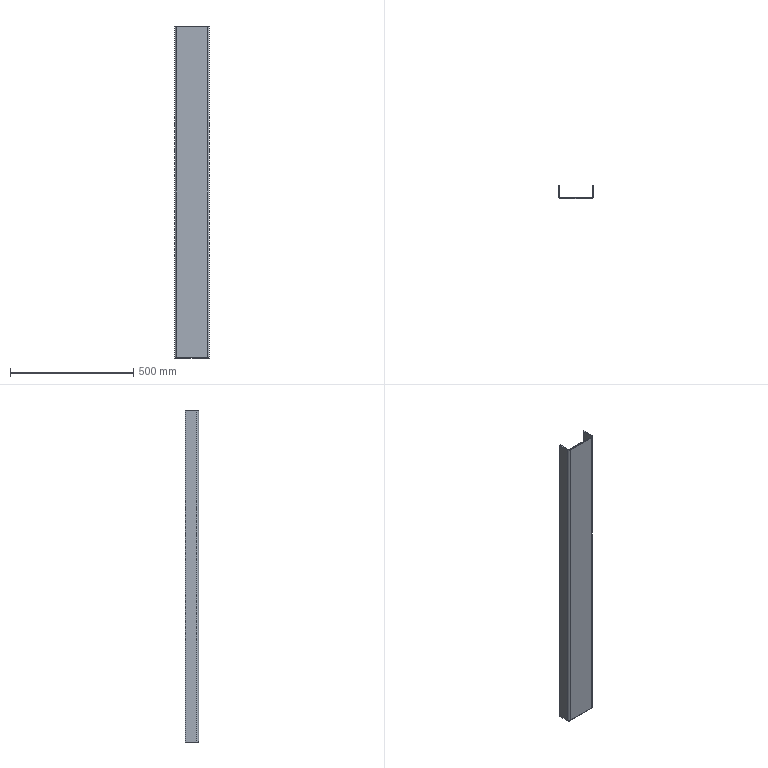Component | SolidWorks | LiftingVerticalBeamAssembly-2_LiftingVerticalBeam-1 | 1 solid | 26 faces | box 140 x 54 x 1345 mm | volume 1257606 mm3 | plane 22 | cylinder 4 | commonest cylinder face diameters 10 x2 18 x2 | material Plain Carbon Steel
STEP:
#1=CARTESIAN_POINT('',(14.893,-1.27,79.625));
#2=VERTEX_POINT('',#1);
#3=CARTESIAN_POINT('',(14.661,-1.27,79.625));
#4=VERTEX_POINT('',#3);
#5=CARTESIAN_POINT('',(14.539,-1.27,79.625));
#6=DIRECTION('',(-1.,0.,0.));
#7=VECTOR('',#6,39.37);
#8=LINE('',#5,#7);
#9=EDGE_CURVE('',#2,#4,#8,.T.);
#10=ORIENTED_EDGE('',*,*,#9,.F.);
#11=CARTESIAN_POINT('',(14.893,-1.199,79.625));
#12=VERTEX_POINT('',#11);
#13=CARTESIAN_POINT('',(14.893,-1.199,79.625));
#14=DIRECTION('',(0.,-1.,0.));
#15=VECTOR('',#14,39.37);
#16=LINE('',#13,#15);
#17=EDGE_CURVE('',#12,#2,#16,.T.);
#18=ORIENTED_EDGE('',*,*,#17,.F.);
#19=CARTESIAN_POINT('',(14.696,-1.002,79.625));
#20=VERTEX_POINT('',#19);
#21=CARTESIAN_POINT('',(14.893,-1.002,79.625));
#22=DIRECTION('',(0.,0.,1.));
#23=DIRECTION('',(1.,0.,0.));
#24=AXIS2_PLACEMENT_3D('',#21,#22,#23);
#25=CIRCLE('',#24,0.1969);
#26=EDGE_CURVE('',#20,#12,#25,.T.);
#27=ORIENTED_EDGE('',*,*,#26,.F.);
#28=CARTESIAN_POINT('',(14.539,-1.002,79.625));
#29=VERTEX_POINT('',#28);
#30=CARTESIAN_POINT('',(14.539,-1.002,79.625));
#31=DIRECTION('',(1.,0.,0.));
#32=VECTOR('',#31,39.37);
#33=LINE('',#30,#32);
#34=EDGE_CURVE('',#29,#20,#33,.T.);
#35=ORIENTED_EDGE('',*,*,#34,.F.);
#36=CARTESIAN_POINT('',(14.893,-1.002,79.625));
#37=DIRECTION('',(0.,0.,1.));
#38=DIRECTION('',(-1.,0.,0.));
#39=AXIS2_PLACEMENT_3D('',#36,#37,#38);
#40=CIRCLE('',#39,0.3543);
#41=EDGE_CURVE('',#29,#4,#40,.T.);
#42=ORIENTED_EDGE('',*,*,#41,.T.);
#43=EDGE_LOOP('',(#10,#18,#27,#35,#42));
#44=FACE_OUTER_BOUND('',#43,.T.);
#45=CARTESIAN_POINT('',(14.539,-1.002,79.625));
#46=DIRECTION('',(0.,0.,1.));
#47=DIRECTION('',(1.,0.,0.));
#48=AXIS2_PLACEMENT_3D('',#45,#46,#47);
#49=PLANE('',#48);
#50=ADVANCED_FACE('',(#44),#49,.T.);
#51=CARTESIAN_POINT('',(14.539,0.7696,79.625));
#52=VERTEX_POINT('',#51);
#53=CARTESIAN_POINT('',(14.539,0.7696,79.625));
#54=DIRECTION('',(0.,-1.,0.));
#55=VECTOR('',#54,39.37);
#56=LINE('',#53,#55);
#57=EDGE_CURVE('',#52,#29,#56,.T.);
#58=ORIENTED_EDGE('',*,*,#57,.T.);
#59=ORIENTED_EDGE('',*,*,#34,.T.);
#60=CARTESIAN_POINT('',(14.696,0.7696,79.625));
#61=VERTEX_POINT('',#60);
#62=CARTESIAN_POINT('',(14.696,0.7696,79.625));
#63=DIRECTION('',(0.,-1.,0.));
#64=VECTOR('',#63,39.37);
#65=LINE('',#62,#64);
#66=EDGE_CURVE('',#61,#20,#65,.T.);
#67=ORIENTED_EDGE('',*,*,#66,.F.);
#68=CARTESIAN_POINT('',(14.539,0.7696,79.625));
#69=DIRECTION('',(1.,0.,0.));
#70=VECTOR('',#69,39.37);
#71=LINE('',#68,#70);
#72=EDGE_CURVE('',#52,#61,#71,.T.);
#73=ORIENTED_EDGE('',*,*,#72,.F.);
#74=EDGE_LOOP('',(#58,#59,#67,#73));
#75=FACE_OUTER_BOUND('',#74,.T.);
#76=CARTESIAN_POINT('',(14.893,-1.199,79.625));
#77=DIRECTION('',(0.,0.,1.));
#78=DIRECTION('',(1.,0.,0.));
#79=AXIS2_PLACEMENT_3D('',#76,#77,#78);
#80=PLANE('',#79);
#81=ADVANCED_FACE('',(#75),#80,.T.);
#82=CARTESIAN_POINT('',(14.661,-1.27,26.672));
#83=VERTEX_POINT('',#82);
#84=CARTESIAN_POINT('',(14.893,-1.27,26.672));
#85=VERTEX_POINT('',#84);
#86=CARTESIAN_POINT('',(14.893,-1.27,26.672));
#87=DIRECTION('',(1.,0.,0.));
#88=VECTOR('',#87,39.37);
#89=LINE('',#86,#88);
#90=EDGE_CURVE('',#83,#85,#89,.T.);
#91=ORIENTED_EDGE('',*,*,#90,.F.);
#92=CARTESIAN_POINT('',(14.539,-1.002,26.672));
#93=VERTEX_POINT('',#92);
#94=CARTESIAN_POINT('',(14.893,-1.002,26.672));
#95=DIRECTION('',(0.,0.,1.));
#96=DIRECTION('',(-1.,0.,0.));
#97=AXIS2_PLACEMENT_3D('',#94,#95,#96);
#98=CIRCLE('',#97,0.3543);
#99=EDGE_CURVE('',#93,#83,#98,.T.);
#100=ORIENTED_EDGE('',*,*,#99,.F.);
#101=CARTESIAN_POINT('',(14.696,-1.002,26.672));
#102=VERTEX_POINT('',#101);
#103=CARTESIAN_POINT('',(14.696,-1.002,26.672));
#104=DIRECTION('',(-1.,0.,0.));
#105=VECTOR('',#104,39.37);
#106=LINE('',#103,#105);
#107=EDGE_CURVE('',#102,#93,#106,.T.);
#108=ORIENTED_EDGE('',*,*,#107,.F.);
#109=CARTESIAN_POINT('',(14.893,-1.199,26.672));
#110=VERTEX_POINT('',#109);
#111=CARTESIAN_POINT('',(14.893,-1.002,26.672));
#112=DIRECTION('',(0.,0.,1.));
#113=DIRECTION('',(1.,0.,0.));
#114=AXIS2_PLACEMENT_3D('',#111,#112,#113);
#115=CIRCLE('',#114,0.1969);
#116=EDGE_CURVE('',#102,#110,#115,.T.);
#117=ORIENTED_EDGE('',*,*,#116,.T.);
#118=CARTESIAN_POINT('',(14.893,-1.356,26.672));
#119=DIRECTION('',(0.,1.,0.));
#120=VECTOR('',#119,39.37);
#121=LINE('',#118,#120);
#122=EDGE_CURVE('',#85,#110,#121,.T.);
#123=ORIENTED_EDGE('',*,*,#122,.F.);
#124=EDGE_LOOP('',(#91,#100,#108,#117,#123));
#125=FACE_OUTER_BOUND('',#124,.T.);
#126=CARTESIAN_POINT('',(14.893,-1.356,26.672));
#127=DIRECTION('',(0.,0.,-1.));
#128=DIRECTION('',(-1.,0.,0.));
#129=AXIS2_PLACEMENT_3D('',#126,#127,#128);
#130=PLANE('',#129);
#131=ADVANCED_FACE('',(#125),#130,.T.);
#132=CARTESIAN_POINT('',(19.696,-1.27,26.672));
#133=VERTEX_POINT('',#132);
#134=CARTESIAN_POINT('',(14.696,-1.27,26.672));
#135=DIRECTION('',(1.,0.,0.));
#136=VECTOR('',#135,39.37);
#137=LINE('',#134,#136);
#138=EDGE_CURVE('',#85,#133,#137,.T.);
#139=ORIENTED_EDGE('',*,*,#138,.F.);
#140=ORIENTED_EDGE('',*,*,#122,.T.);
#141=CARTESIAN_POINT('',(19.696,-1.199,26.672));
#142=VERTEX_POINT('',#141);
#143=CARTESIAN_POINT('',(14.539,-1.199,26.672));
#144=DIRECTION('',(1.,0.,0.));
#145=VECTOR('',#144,39.37);
#146=LINE('',#143,#145);
#147=EDGE_CURVE('',#110,#142,#146,.T.);
#148=ORIENTED_EDGE('',*,*,#147,.T.);
#149=CARTESIAN_POINT('',(19.696,-1.199,26.672));
#150=DIRECTION('',(0.,-1.,0.));
#151=VECTOR('',#150,39.37);
#152=LINE('',#149,#151);
#153=EDGE_CURVE('',#142,#133,#152,.T.);
#154=ORIENTED_EDGE('',*,*,#153,.T.);
#155=EDGE_LOOP('',(#139,#140,#148,#154));
#156=FACE_OUTER_BOUND('',#155,.T.);
#157=CARTESIAN_POINT('',(14.696,-1.002,26.672));
#158=DIRECTION('',(0.,0.,-1.));
#159=DIRECTION('',(-1.,0.,0.));
#160=AXIS2_PLACEMENT_3D('',#157,#158,#159);
#161=PLANE('',#160);
#162=ADVANCED_FACE('',(#156),#161,.T.);
#163=CARTESIAN_POINT('',(19.929,-1.27,79.625));
#164=VERTEX_POINT('',#163);
#165=CARTESIAN_POINT('',(19.696,-1.27,79.625));
#166=VERTEX_POINT('',#165);
#167=CARTESIAN_POINT('',(19.696,-1.27,79.625));
#168=DIRECTION('',(-1.,0.,0.));
#169=VECTOR('',#168,39.37);
#170=LINE('',#167,#169);
#171=EDGE_CURVE('',#164,#166,#170,.T.);
#172=ORIENTED_EDGE('',*,*,#171,.F.);
#173=CARTESIAN_POINT('',(20.051,-1.002,79.625));
#174=VERTEX_POINT('',#173);
#175=CARTESIAN_POINT('',(19.696,-1.002,79.625));
#176=DIRECTION('',(0.,0.,1.));
#177=DIRECTION('',(-1.,-0.,0.));
#178=AXIS2_PLACEMENT_3D('',#175,#176,#177);
#179=CIRCLE('',#178,0.3543);
#180=EDGE_CURVE('',#164,#174,#179,.T.);
#181=ORIENTED_EDGE('',*,*,#180,.T.);
#182=CARTESIAN_POINT('',(19.893,-1.002,79.625));
#183=VERTEX_POINT('',#182);
#184=CARTESIAN_POINT('',(19.893,-1.002,79.625));
#185=DIRECTION('',(1.,0.,0.));
#186=VECTOR('',#185,39.37);
#187=LINE('',#184,#186);
#188=EDGE_CURVE('',#183,#174,#187,.T.);
#189=ORIENTED_EDGE('',*,*,#188,.F.);
#190=CARTESIAN_POINT('',(19.696,-1.199,79.625));
#191=VERTEX_POINT('',#190);
#192=CARTESIAN_POINT('',(19.696,-1.002,79.625));
#193=DIRECTION('',(0.,0.,1.));
#194=DIRECTION('',(1.,0.,0.));
#195=AXIS2_PLACEMENT_3D('',#192,#193,#194);
#196=CIRCLE('',#195,0.1969);
#197=EDGE_CURVE('',#191,#183,#196,.T.);
#198=ORIENTED_EDGE('',*,*,#197,.F.);
#199=CARTESIAN_POINT('',(19.696,-1.356,79.625));
#200=DIRECTION('',(0.,1.,0.));
#201=VECTOR('',#200,39.37);
#202=LINE('',#199,#201);
#203=EDGE_CURVE('',#166,#191,#202,.T.);
#204=ORIENTED_EDGE('',*,*,#203,.F.);
#205=EDGE_LOOP('',(#172,#181,#189,#198,#204));
#206=FACE_OUTER_BOUND('',#205,.T.);
#207=CARTESIAN_POINT('',(19.696,-1.356,79.625));
#208=DIRECTION('',(0.,0.,1.));
#209=DIRECTION('',(1.,0.,0.));
#210=AXIS2_PLACEMENT_3D('',#207,#208,#209);
#211=PLANE('',#210);
#212=ADVANCED_FACE('',(#206),#211,.T.);
#213=CARTESIAN_POINT('',(19.893,-1.27,79.625));
#214=DIRECTION('',(-1.,0.,0.));
#215=VECTOR('',#214,39.37);
#216=LINE('',#213,#215);
#217=EDGE_CURVE('',#166,#2,#216,.T.);
#218=ORIENTED_EDGE('',*,*,#217,.F.);
#219=ORIENTED_EDGE('',*,*,#203,.T.);
#220=CARTESIAN_POINT('',(14.539,-1.199,79.625));
#221=DIRECTION('',(1.,0.,0.));
#222=VECTOR('',#221,39.37);
#223=LINE('',#220,#222);
#224=EDGE_CURVE('',#12,#191,#223,.T.);
#225=ORIENTED_EDGE('',*,*,#224,.F.);
#226=ORIENTED_EDGE('',*,*,#17,.T.);
#227=EDGE_LOOP('',(#218,#219,#225,#226));
#228=FACE_OUTER_BOUND('',#227,.T.);
#229=CARTESIAN_POINT('',(19.893,-1.002,79.625));
#230=DIRECTION('',(0.,0.,1.));
#231=DIRECTION('',(1.,0.,0.));
#232=AXIS2_PLACEMENT_3D('',#229,#230,#231);
#233=PLANE('',#232);
#234=ADVANCED_FACE('',(#228),#233,.T.);
#235=CARTESIAN_POINT('',(19.929,-1.27,26.672));
#236=VERTEX_POINT('',#235);
#237=CARTESIAN_POINT('',(20.051,-1.27,26.672));
#238=DIRECTION('',(1.,0.,0.));
#239=VECTOR('',#238,39.37);
#240=LINE('',#237,#239);
#241=EDGE_CURVE('',#133,#236,#240,.T.);
#242=ORIENTED_EDGE('',*,*,#241,.F.);
#243=ORIENTED_EDGE('',*,*,#153,.F.);
#244=CARTESIAN_POINT('',(19.893,-1.002,26.672));
#245=VERTEX_POINT('',#244);
#246=CARTESIAN_POINT('',(19.696,-1.002,26.672));
#247=DIRECTION('',(0.,0.,1.));
#248=DIRECTION('',(1.,0.,0.));
#249=AXIS2_PLACEMENT_3D('',#246,#247,#248);
#250=CIRCLE('',#249,0.1969);
#251=EDGE_CURVE('',#142,#245,#250,.T.);
#252=ORIENTED_EDGE('',*,*,#251,.T.);
#253=CARTESIAN_POINT('',(20.051,-1.002,26.672));
#254=VERTEX_POINT('',#253);
#255=CARTESIAN_POINT('',(20.051,-1.002,26.672));
#256=DIRECTION('',(-1.,0.,0.));
#257=VECTOR('',#256,39.37);
#258=LINE('',#255,#257);
#259=EDGE_CURVE('',#254,#245,#258,.T.);
#260=ORIENTED_EDGE('',*,*,#259,.F.);
#261=CARTESIAN_POINT('',(19.696,-1.002,26.672));
#262=DIRECTION('',(0.,0.,1.));
#263=DIRECTION('',(-1.,-0.,0.));
#264=AXIS2_PLACEMENT_3D('',#261,#262,#263);
#265=CIRCLE('',#264,0.3543);
#266=EDGE_CURVE('',#236,#254,#265,.T.);
#267=ORIENTED_EDGE('',*,*,#266,.F.);
#268=EDGE_LOOP('',(#242,#243,#252,#260,#267));
#269=FACE_OUTER_BOUND('',#268,.T.);
#270=CARTESIAN_POINT('',(20.051,-1.002,26.672));
#271=DIRECTION('',(0.,0.,-1.));
#272=DIRECTION('',(-1.,0.,0.));
#273=AXIS2_PLACEMENT_3D('',#270,#271,#272);
#274=PLANE('',#273);
#275=ADVANCED_FACE('',(#269),#274,.T.);
#276=CARTESIAN_POINT('',(20.051,0.7696,26.672));
#277=VERTEX_POINT('',#276);
#278=CARTESIAN_POINT('',(20.051,-1.356,26.672));
#279=DIRECTION('',(0.,1.,0.));
#280=VECTOR('',#279,39.37);
#281=LINE('',#278,#280);
#282=EDGE_CURVE('',#254,#277,#281,.T.);
#283=ORIENTED_EDGE('',*,*,#282,.F.);
#284=ORIENTED_EDGE('',*,*,#259,.T.);
#285=CARTESIAN_POINT('',(19.893,0.7696,26.672));
#286=VERTEX_POINT('',#285);
#287=CARTESIAN_POINT('',(19.893,-1.356,26.672));
#288=DIRECTION('',(0.,1.,0.));
#289=VECTOR('',#288,39.37);
#290=LINE('',#287,#289);
#291=EDGE_CURVE('',#245,#286,#290,.T.);
#292=ORIENTED_EDGE('',*,*,#291,.T.);
#293=CARTESIAN_POINT('',(19.893,0.7696,26.672));
#294=DIRECTION('',(1.,0.,0.));
#295=VECTOR('',#294,39.37);
#296=LINE('',#293,#295);
#297=EDGE_CURVE('',#286,#277,#296,.T.);
#298=ORIENTED_EDGE('',*,*,#297,.T.);
#299=EDGE_LOOP('',(#283,#284,#292,#298));
#300=FACE_OUTER_BOUND('',#299,.T.);
#301=CARTESIAN_POINT('',(19.696,-1.199,26.672));
#302=DIRECTION('',(0.,0.,-1.));
#303=DIRECTION('',(-1.,0.,0.));
#304=AXIS2_PLACEMENT_3D('',#301,#302,#303);
#305=PLANE('',#304);
#306=ADVANCED_FACE('',(#300),#305,.T.);
#307=ORIENTED_EDGE('',*,*,#282,.T.);
#308=CARTESIAN_POINT('',(20.051,0.7696,79.625));
#309=VERTEX_POINT('',#308);
#310=CARTESIAN_POINT('',(20.051,0.7696,79.625));
#311=DIRECTION('',(0.,0.,-1.));
#312=VECTOR('',#311,39.37);
#313=LINE('',#310,#312);
#314=EDGE_CURVE('',#309,#277,#313,.T.);
#315=ORIENTED_EDGE('',*,*,#314,.F.);
#316=CARTESIAN_POINT('',(20.051,-1.356,79.625));
#317=DIRECTION('',(0.,1.,0.));
#318=VECTOR('',#317,39.37);
#319=LINE('',#316,#318);
#320=EDGE_CURVE('',#174,#309,#319,.T.);
#321=ORIENTED_EDGE('',*,*,#320,.F.);
#322=CARTESIAN_POINT('',(20.051,-1.002,79.625));
#323=DIRECTION('',(0.,0.,-1.));
#324=VECTOR('',#323,39.37);
#325=LINE('',#322,#324);
#326=EDGE_CURVE('',#174,#254,#325,.T.);
#327=ORIENTED_EDGE('',*,*,#326,.T.);
#328=EDGE_LOOP('',(#307,#315,#321,#327));
#329=FACE_OUTER_BOUND('',#328,.T.);
#330=CARTESIAN_POINT('',(20.051,-1.356,79.625));
#331=DIRECTION('',(-1.,0.,0.));
#332=DIRECTION('',(0.,0.,1.));
#333=AXIS2_PLACEMENT_3D('',#330,#331,#332);
#334=PLANE('',#333);
#335=ADVANCED_FACE('',(#329),#334,.F.);
#336=ORIENTED_EDGE('',*,*,#297,.F.);
#337=CARTESIAN_POINT('',(19.893,0.7696,79.625));
#338=VERTEX_POINT('',#337);
#339=CARTESIAN_POINT('',(19.893,0.7696,79.625));
#340=DIRECTION('',(0.,0.,-1.));
#341=VECTOR('',#340,39.37);
#342=LINE('',#339,#341);
#343=EDGE_CURVE('',#338,#286,#342,.T.);
#344=ORIENTED_EDGE('',*,*,#343,.F.);
#345=CARTESIAN_POINT('',(19.893,0.7696,79.625));
#346=DIRECTION('',(1.,0.,0.));
#347=VECTOR('',#346,39.37);
#348=LINE('',#345,#347);
#349=EDGE_CURVE('',#338,#309,#348,.T.);
#350=ORIENTED_EDGE('',*,*,#349,.T.);
#351=ORIENTED_EDGE('',*,*,#314,.T.);
#352=EDGE_LOOP('',(#336,#344,#350,#351));
#353=FACE_OUTER_BOUND('',#352,.T.);
#354=CARTESIAN_POINT('',(19.893,0.7696,79.625));
#355=DIRECTION('',(0.,1.,0.));
#356=DIRECTION('',(0.,0.,1.));
#357=AXIS2_PLACEMENT_3D('',#354,#355,#356);
#358=PLANE('',#357);
#359=ADVANCED_FACE('',(#353),#358,.T.);
#360=ORIENTED_EDGE('',*,*,#291,.F.);
#361=CARTESIAN_POINT('',(19.893,-1.002,79.625));
#362=DIRECTION('',(0.,0.,-1.));
#363=VECTOR('',#362,39.37);
#364=LINE('',#361,#363);
#365=EDGE_CURVE('',#183,#245,#364,.T.);
#366=ORIENTED_EDGE('',*,*,#365,.F.);
#367=CARTESIAN_POINT('',(19.893,-1.356,79.625));
#368=DIRECTION('',(0.,1.,0.));
#369=VECTOR('',#368,39.37);
#370=LINE('',#367,#369);
#371=EDGE_CURVE('',#183,#338,#370,.T.);
#372=ORIENTED_EDGE('',*,*,#371,.T.);
#373=ORIENTED_EDGE('',*,*,#343,.T.);
#374=EDGE_LOOP('',(#360,#366,#372,#373));
#375=FACE_OUTER_BOUND('',#374,.T.);
#376=CARTESIAN_POINT('',(19.893,-1.356,79.625));
#377=DIRECTION('',(-1.,0.,0.));
#378=DIRECTION('',(0.,0.,1.));
#379=AXIS2_PLACEMENT_3D('',#376,#377,#378);
#380=PLANE('',#379);
#381=ADVANCED_FACE('',(#375),#380,.T.);
#382=ORIENTED_EDGE('',*,*,#251,.F.);
#383=CARTESIAN_POINT('',(19.696,-1.199,79.625));
#384=DIRECTION('',(0.,0.,-1.));
#385=VECTOR('',#384,39.37);
#386=LINE('',#383,#385);
#387=EDGE_CURVE('',#191,#142,#386,.T.);
#388=ORIENTED_EDGE('',*,*,#387,.F.);
#389=ORIENTED_EDGE('',*,*,#197,.T.);
#390=ORIENTED_EDGE('',*,*,#365,.T.);
#391=EDGE_LOOP('',(#382,#388,#389,#390));
#392=FACE_OUTER_BOUND('',#391,.T.);
#393=CARTESIAN_POINT('',(19.696,-1.002,79.625));
#394=DIRECTION('',(0.,0.,-1.));
#395=DIRECTION('',(-1.,0.,0.));
#396=AXIS2_PLACEMENT_3D('',#393,#394,#395);
#397=CYLINDRICAL_SURFACE('',#396,0.1969);
#398=ADVANCED_FACE('',(#392),#397,.F.);
#399=ORIENTED_EDGE('',*,*,#147,.F.);
#400=CARTESIAN_POINT('',(14.893,-1.199,79.625));
#401=DIRECTION('',(0.,0.,-1.));
#402=VECTOR('',#401,39.37);
#403=LINE('',#400,#402);
#404=EDGE_CURVE('',#12,#110,#403,.T.);
#405=ORIENTED_EDGE('',*,*,#404,.F.);
#406=ORIENTED_EDGE('',*,*,#224,.T.);
#407=ORIENTED_EDGE('',*,*,#387,.T.);
#408=EDGE_LOOP('',(#399,#405,#406,#407));
#409=FACE_OUTER_BOUND('',#408,.T.);
#410=CARTESIAN_POINT('',(14.539,-1.199,79.625));
#411=DIRECTION('',(0.,1.,0.));
#412=DIRECTION('',(0.,0.,1.));
#413=AXIS2_PLACEMENT_3D('',#410,#411,#412);
#414=PLANE('',#413);
#415=ADVANCED_FACE('',(#409),#414,.T.);
#416=ORIENTED_EDGE('',*,*,#116,.F.);
#417=CARTESIAN_POINT('',(14.696,-1.002,79.625));
#418=DIRECTION('',(0.,0.,-1.));
#419=VECTOR('',#418,39.37);
#420=LINE('',#417,#419);
#421=EDGE_CURVE('',#20,#102,#420,.T.);
#422=ORIENTED_EDGE('',*,*,#421,.F.);
#423=ORIENTED_EDGE('',*,*,#26,.T.);
#424=ORIENTED_EDGE('',*,*,#404,.T.);
#425=EDGE_LOOP('',(#416,#422,#423,#424));
#426=FACE_OUTER_BOUND('',#425,.T.);
#427=CARTESIAN_POINT('',(14.893,-1.002,79.625));
#428=DIRECTION('',(0.,0.,-1.));
#429=DIRECTION('',(-1.,0.,0.));
#430=AXIS2_PLACEMENT_3D('',#427,#428,#429);
#431=CYLINDRICAL_SURFACE('',#430,0.1969);
#432=ADVANCED_FACE('',(#426),#431,.F.);
#433=CARTESIAN_POINT('',(14.696,0.7696,26.672));
#434=VERTEX_POINT('',#433);
#435=CARTESIAN_POINT('',(14.696,0.7696,26.672));
#436=DIRECTION('',(0.,-1.,0.));
#437=VECTOR('',#436,39.37);
#438=LINE('',#435,#437);
#439=EDGE_CURVE('',#434,#102,#438,.T.);
#440=ORIENTED_EDGE('',*,*,#439,.F.);
#441=CARTESIAN_POINT('',(14.696,0.7696,79.625));
#442=DIRECTION('',(0.,0.,-1.));
#443=VECTOR('',#442,39.37);
#444=LINE('',#441,#443);
#445=EDGE_CURVE('',#61,#434,#444,.T.);
#446=ORIENTED_EDGE('',*,*,#445,.F.);
#447=ORIENTED_EDGE('',*,*,#66,.T.);
#448=ORIENTED_EDGE('',*,*,#421,.T.);
#449=EDGE_LOOP('',(#440,#446,#447,#448));
#450=FACE_OUTER_BOUND('',#449,.T.);
#451=CARTESIAN_POINT('',(14.696,0.7696,79.625));
#452=DIRECTION('',(1.,0.,0.));
#453=DIRECTION('',(-0.,1.,0.));
#454=AXIS2_PLACEMENT_3D('',#451,#452,#453);
#455=PLANE('',#454);
#456=ADVANCED_FACE('',(#450),#455,.T.);
#457=CARTESIAN_POINT('',(14.539,0.7696,26.672));
#458=VERTEX_POINT('',#457);
#459=CARTESIAN_POINT('',(14.539,0.7696,26.672));
#460=DIRECTION('',(1.,0.,0.));
#461=VECTOR('',#460,39.37);
#462=LINE('',#459,#461);
#463=EDGE_CURVE('',#458,#434,#462,.T.);
#464=ORIENTED_EDGE('',*,*,#463,.F.);
#465=CARTESIAN_POINT('',(14.539,0.7696,79.625));
#466=DIRECTION('',(0.,0.,-1.));
#467=VECTOR('',#466,39.37);
#468=LINE('',#465,#467);
#469=EDGE_CURVE('',#52,#458,#468,.T.);
#470=ORIENTED_EDGE('',*,*,#469,.F.);
#471=ORIENTED_EDGE('',*,*,#72,.T.);
#472=ORIENTED_EDGE('',*,*,#445,.T.);
#473=EDGE_LOOP('',(#464,#470,#471,#472));
#474=FACE_OUTER_BOUND('',#473,.T.);
#475=CARTESIAN_POINT('',(14.539,0.7696,79.625));
#476=DIRECTION('',(-0.,1.,0.));
#477=DIRECTION('',(-1.,-0.,0.));
#478=AXIS2_PLACEMENT_3D('',#475,#476,#477);
#479=PLANE('',#478);
#480=ADVANCED_FACE('',(#474),#479,.T.);
#481=CARTESIAN_POINT('',(14.539,0.7696,26.672));
#482=DIRECTION('',(0.,-1.,0.));
#483=VECTOR('',#482,39.37);
#484=LINE('',#481,#483);
#485=EDGE_CURVE('',#458,#93,#484,.T.);
#486=ORIENTED_EDGE('',*,*,#485,.T.);
#487=CARTESIAN_POINT('',(14.539,-1.002,79.625));
#488=DIRECTION('',(0.,0.,-1.));
#489=VECTOR('',#488,39.37);
#490=LINE('',#487,#489);
#491=EDGE_CURVE('',#29,#93,#490,.T.);
#492=ORIENTED_EDGE('',*,*,#491,.F.);
#493=ORIENTED_EDGE('',*,*,#57,.F.);
#494=ORIENTED_EDGE('',*,*,#469,.T.);
#495=EDGE_LOOP('',(#486,#492,#493,#494));
#496=FACE_OUTER_BOUND('',#495,.T.);
#497=CARTESIAN_POINT('',(14.539,0.7696,79.625));
#498=DIRECTION('',(1.,0.,0.));
#499=DIRECTION('',(-0.,1.,0.));
#500=AXIS2_PLACEMENT_3D('',#497,#498,#499);
#501=PLANE('',#500);
#502=ADVANCED_FACE('',(#496),#501,.F.);
#503=CARTESIAN_POINT('',(14.893,-1.356,79.538));
#504=VERTEX_POINT('',#503);
#505=CARTESIAN_POINT('',(14.893,-1.356,26.759));
#506=VERTEX_POINT('',#505);
#507=CARTESIAN_POINT('',(14.893,-1.356,79.625));
#508=DIRECTION('',(0.,0.,-1.));
#509=VECTOR('',#508,39.37);
#510=LINE('',#507,#509);
#511=EDGE_CURVE('',#504,#506,#510,.T.);
#512=ORIENTED_EDGE('',*,*,#511,.F.);
#513=CARTESIAN_POINT('',(14.661,-1.27,79.538));
#514=VERTEX_POINT('',#513);
#515=CARTESIAN_POINT('',(14.893,-1.002,79.538));
#516=DIRECTION('',(0.,0.,-1.));
#517=DIRECTION('',(-1.,0.,0.));
#518=AXIS2_PLACEMENT_3D('',#515,#516,#517);
#519=CIRCLE('',#518,0.3543);
#520=EDGE_CURVE('',#504,#514,#519,.T.);
#521=ORIENTED_EDGE('',*,*,#520,.T.);
#522=CARTESIAN_POINT('',(14.661,-1.27,79.625));
#523=DIRECTION('',(0.,0.,1.));
#524=VECTOR('',#523,39.37);
#525=LINE('',#522,#524);
#526=EDGE_CURVE('',#514,#4,#525,.T.);
#527=ORIENTED_EDGE('',*,*,#526,.T.);
#528=ORIENTED_EDGE('',*,*,#41,.F.);
#529=ORIENTED_EDGE('',*,*,#491,.T.);
#530=ORIENTED_EDGE('',*,*,#99,.T.);
#531=CARTESIAN_POINT('',(14.661,-1.27,26.759));
#532=VERTEX_POINT('',#531);
#533=CARTESIAN_POINT('',(14.661,-1.27,79.625));
#534=DIRECTION('',(0.,0.,1.));
#535=VECTOR('',#534,39.37);
#536=LINE('',#533,#535);
#537=EDGE_CURVE('',#83,#532,#536,.T.);
#538=ORIENTED_EDGE('',*,*,#537,.T.);
#539=CARTESIAN_POINT('',(14.893,-1.002,26.759));
#540=DIRECTION('',(0.,0.,1.));
#541=DIRECTION('',(1.,0.,0.));
#542=AXIS2_PLACEMENT_3D('',#539,#540,#541);
#543=CIRCLE('',#542,0.3543);
#544=EDGE_CURVE('',#532,#506,#543,.T.);
#545=ORIENTED_EDGE('',*,*,#544,.T.);
#546=EDGE_LOOP('',(#512,#521,#527,#528,#529,#530,#538,#545));
#547=FACE_OUTER_BOUND('',#546,.T.);
#548=CARTESIAN_POINT('',(14.893,-1.002,79.625));
#549=DIRECTION('',(0.,0.,-1.));
#550=DIRECTION('',(-1.,0.,0.));
#551=AXIS2_PLACEMENT_3D('',#548,#549,#550);
#552=CYLINDRICAL_SURFACE('',#551,0.3543);
#553=ADVANCED_FACE('',(#547),#552,.T.);
#554=CARTESIAN_POINT('',(19.696,-1.356,79.538));
#555=VERTEX_POINT('',#554);
#556=CARTESIAN_POINT('',(19.696,-1.356,26.759));
#557=VERTEX_POINT('',#556);
#558=CARTESIAN_POINT('',(19.696,-1.356,79.625));
#559=DIRECTION('',(0.,0.,-1.));
#560=VECTOR('',#559,39.37);
#561=LINE('',#558,#560);
#562=EDGE_CURVE('',#555,#557,#561,.T.);
#563=ORIENTED_EDGE('',*,*,#562,.F.);
#564=CARTESIAN_POINT('',(14.539,-1.356,79.538));
#565=DIRECTION('',(-1.,0.,0.));
#566=VECTOR('',#565,39.37);
#567=LINE('',#564,#566);
#568=EDGE_CURVE('',#555,#504,#567,.T.);
#569=ORIENTED_EDGE('',*,*,#568,.T.);
#570=ORIENTED_EDGE('',*,*,#511,.T.);
#571=CARTESIAN_POINT('',(14.539,-1.356,26.759));
#572=DIRECTION('',(1.,0.,0.));
#573=VECTOR('',#572,39.37);
#574=LINE('',#571,#573);
#575=EDGE_CURVE('',#506,#557,#574,.T.);
#576=ORIENTED_EDGE('',*,*,#575,.T.);
#577=EDGE_LOOP('',(#563,#569,#570,#576));
#578=FACE_OUTER_BOUND('',#577,.T.);
#579=CARTESIAN_POINT('',(14.539,-1.356,79.625));
#580=DIRECTION('',(0.,1.,0.));
#581=DIRECTION('',(0.,0.,1.));
#582=AXIS2_PLACEMENT_3D('',#579,#580,#581);
#583=PLANE('',#582);
#584=ADVANCED_FACE('',(#578),#583,.F.);
#585=CARTESIAN_POINT('',(19.929,-1.27,79.538));
#586=VERTEX_POINT('',#585);
#587=CARTESIAN_POINT('',(19.929,-1.27,79.625));
#588=DIRECTION('',(0.,0.,-1.));
#589=VECTOR('',#588,39.37);
#590=LINE('',#587,#589);
#591=EDGE_CURVE('',#164,#586,#590,.T.);
#592=ORIENTED_EDGE('',*,*,#591,.T.);
#593=CARTESIAN_POINT('',(19.696,-1.002,79.538));
#594=DIRECTION('',(0.,0.,-1.));
#595=DIRECTION('',(-1.,0.,0.));
#596=AXIS2_PLACEMENT_3D('',#593,#594,#595);
#597=CIRCLE('',#596,0.3543);
#598=EDGE_CURVE('',#586,#555,#597,.T.);
#599=ORIENTED_EDGE('',*,*,#598,.T.);
#600=ORIENTED_EDGE('',*,*,#562,.T.);
#601=CARTESIAN_POINT('',(19.929,-1.27,26.759));
#602=VERTEX_POINT('',#601);
#603=CARTESIAN_POINT('',(19.696,-1.002,26.759));
#604=DIRECTION('',(0.,0.,1.));
#605=DIRECTION('',(1.,0.,0.));
#606=AXIS2_PLACEMENT_3D('',#603,#604,#605);
#607=CIRCLE('',#606,0.3543);
#608=EDGE_CURVE('',#557,#602,#607,.T.);
#609=ORIENTED_EDGE('',*,*,#608,.T.);
#610=CARTESIAN_POINT('',(19.929,-1.27,79.625));
#611=DIRECTION('',(0.,0.,-1.));
#612=VECTOR('',#611,39.37);
#613=LINE('',#610,#612);
#614=EDGE_CURVE('',#602,#236,#613,.T.);
#615=ORIENTED_EDGE('',*,*,#614,.T.);
#616=ORIENTED_EDGE('',*,*,#266,.T.);
#617=ORIENTED_EDGE('',*,*,#326,.F.);
#618=ORIENTED_EDGE('',*,*,#180,.F.);
#619=EDGE_LOOP('',(#592,#599,#600,#609,#615,#616,#617,#618));
#620=FACE_OUTER_BOUND('',#619,.T.);
#621=CARTESIAN_POINT('',(19.696,-1.002,79.625));
#622=DIRECTION('',(0.,0.,-1.));
#623=DIRECTION('',(-1.,0.,0.));
#624=AXIS2_PLACEMENT_3D('',#621,#622,#623);
#625=CYLINDRICAL_SURFACE('',#624,0.3543);
#626=ADVANCED_FACE('',(#620),#625,.T.);
#627=ORIENTED_EDGE('',*,*,#320,.T.);
#628=ORIENTED_EDGE('',*,*,#349,.F.);
#629=ORIENTED_EDGE('',*,*,#371,.F.);
#630=ORIENTED_EDGE('',*,*,#188,.T.);
#631=EDGE_LOOP('',(#627,#628,#629,#630));
#632=FACE_OUTER_BOUND('',#631,.T.);
#633=CARTESIAN_POINT('',(19.696,-1.002,79.625));
#634=DIRECTION('',(0.,0.,1.));
#635=DIRECTION('',(1.,0.,0.));
#636=AXIS2_PLACEMENT_3D('',#633,#634,#635);
#637=PLANE('',#636);
#638=ADVANCED_FACE('',(#632),#637,.T.);
#639=ORIENTED_EDGE('',*,*,#439,.T.);
#640=ORIENTED_EDGE('',*,*,#107,.T.);
#641=ORIENTED_EDGE('',*,*,#485,.F.);
#642=ORIENTED_EDGE('',*,*,#463,.T.);
#643=EDGE_LOOP('',(#639,#640,#641,#642));
#644=FACE_OUTER_BOUND('',#643,.T.);
#645=CARTESIAN_POINT('',(19.696,-1.002,26.672));
#646=DIRECTION('',(0.,0.,1.));
#647=DIRECTION('',(1.,0.,0.));
#648=AXIS2_PLACEMENT_3D('',#645,#646,#647);
#649=PLANE('',#648);
#650=ADVANCED_FACE('',(#644),#649,.F.);
#651=ORIENTED_EDGE('',*,*,#9,.T.);
#652=ORIENTED_EDGE('',*,*,#526,.F.);
#653=CARTESIAN_POINT('',(14.539,-1.27,79.538));
#654=DIRECTION('',(1.,0.,0.));
#655=VECTOR('',#654,39.37);
#656=LINE('',#653,#655);
#657=EDGE_CURVE('',#514,#586,#656,.T.);
#658=ORIENTED_EDGE('',*,*,#657,.T.);
#659=ORIENTED_EDGE('',*,*,#591,.F.);
#660=ORIENTED_EDGE('',*,*,#171,.T.);
#661=ORIENTED_EDGE('',*,*,#217,.T.);
#662=EDGE_LOOP('',(#651,#652,#658,#659,#660,#661));
#663=FACE_OUTER_BOUND('',#662,.T.);
#664=CARTESIAN_POINT('',(14.539,-1.27,79.578));
#665=DIRECTION('',(0.,1.,0.));
#666=DIRECTION('',(0.,0.,1.));
#667=AXIS2_PLACEMENT_3D('',#664,#665,#666);
#668=PLANE('',#667);
#669=ADVANCED_FACE('',(#663),#668,.F.);
#670=CARTESIAN_POINT('',(14.539,-1.27,26.759));
#671=DIRECTION('',(1.,0.,0.));
#672=VECTOR('',#671,39.37);
#673=LINE('',#670,#672);
#674=EDGE_CURVE('',#532,#602,#673,.T.);
#675=ORIENTED_EDGE('',*,*,#674,.T.);
#676=ORIENTED_EDGE('',*,*,#608,.F.);
#677=ORIENTED_EDGE('',*,*,#575,.F.);
#678=ORIENTED_EDGE('',*,*,#544,.F.);
#679=EDGE_LOOP('',(#675,#676,#677,#678));
#680=FACE_OUTER_BOUND('',#679,.T.);
#681=CARTESIAN_POINT('',(14.539,-1.386,26.759));
#682=DIRECTION('',(0.,0.,1.));
#683=DIRECTION('',(1.,0.,0.));
#684=AXIS2_PLACEMENT_3D('',#681,#682,#683);
#685=PLANE('',#684);
#686=ADVANCED_FACE('',(#680),#685,.F.);
#687=ORIENTED_EDGE('',*,*,#90,.T.);
#688=ORIENTED_EDGE('',*,*,#138,.T.);
#689=ORIENTED_EDGE('',*,*,#241,.T.);
#690=ORIENTED_EDGE('',*,*,#614,.F.);
#691=ORIENTED_EDGE('',*,*,#674,.F.);
#692=ORIENTED_EDGE('',*,*,#537,.F.);
#693=EDGE_LOOP('',(#687,#688,#689,#690,#691,#692));
#694=FACE_OUTER_BOUND('',#693,.T.);
#695=CARTESIAN_POINT('',(14.539,-1.27,26.634));
#696=DIRECTION('',(0.,1.,0.));
#697=DIRECTION('',(0.,0.,1.));
#698=AXIS2_PLACEMENT_3D('',#695,#696,#697);
#699=PLANE('',#698);
#700=ADVANCED_FACE('',(#694),#699,.F.);
#701=ORIENTED_EDGE('',*,*,#568,.F.);
#702=ORIENTED_EDGE('',*,*,#598,.F.);
#703=ORIENTED_EDGE('',*,*,#657,.F.);
#704=ORIENTED_EDGE('',*,*,#520,.F.);
#705=EDGE_LOOP('',(#701,#702,#703,#704));
#706=FACE_OUTER_BOUND('',#705,.T.);
#707=CARTESIAN_POINT('',(14.539,-1.386,79.538));
#708=DIRECTION('',(0.,0.,-1.));
#709=DIRECTION('',(-1.,0.,0.));
#710=AXIS2_PLACEMENT_3D('',#707,#708,#709);
#711=PLANE('',#710);
#712=ADVANCED_FACE('',(#706),#711,.F.);
#713=CLOSED_SHELL('',(#50,#81,#131,#162,#212,#234,#275,#306,#335,#359,#381,#398,#415,#432,#456,#480,#502,#553,#584,#626,#638,#650,#669,#686,#700,#712));
#714=MANIFOLD_SOLID_BREP('',#713);
#715=CARTESIAN_POINT('',(0.,0.,0.));
#716=DIRECTION('',(0.,0.,1.));
#717=DIRECTION('',(1.,0.,0.));
#718=AXIS2_PLACEMENT_3D('',#715,#716,#717);
#719=(LENGTH_UNIT()NAMED_UNIT(*)SI_UNIT($,.METRE.));
#720=LENGTH_MEASURE_WITH_UNIT(LENGTH_MEASURE(0.0254),#719);
#721=DIMENSIONAL_EXPONENTS(1.,0.,0.,0.,0.,0.,0.);
#722=(CONVERSION_BASED_UNIT('',#720)LENGTH_UNIT()NAMED_UNIT(#721));
#723=UNCERTAINTY_MEASURE_WITH_UNIT(LENGTH_MEASURE(0.00001),#722,'','');
#724=(NAMED_UNIT(*)PLANE_ANGLE_UNIT()SI_UNIT($,.RADIAN.));
#725=(NAMED_UNIT(*)SI_UNIT($,.STERADIAN.)SOLID_ANGLE_UNIT());
#726=(GEOMETRIC_REPRESENTATION_CONTEXT(3)GLOBAL_UNCERTAINTY_ASSIGNED_CONTEXT((#723))GLOBAL_UNIT_ASSIGNED_CONTEXT((#722,#724,#725))REPRESENTATION_CONTEXT('',''));
#727=ADVANCED_BREP_SHAPE_REPRESENTATION('',(#714,#718),#726);
#728=COLOUR_RGB('',0.7922,0.8196,0.9333);
#729=FILL_AREA_STYLE_COLOUR('',#728);
#730=FILL_AREA_STYLE('',(#729));
#731=SURFACE_STYLE_FILL_AREA(#730);
#732=SURFACE_SIDE_STYLE('',(#731));
#733=SURFACE_STYLE_USAGE(.BOTH.,#732);
#734=PRESENTATION_STYLE_ASSIGNMENT((#733));
#735=STYLED_ITEM('',(#734),#714);
#736=(LENGTH_UNIT()NAMED_UNIT(*)SI_UNIT($,.METRE.));
#737=LENGTH_MEASURE_WITH_UNIT(LENGTH_MEASURE(0.0254),#736);
#738=DIMENSIONAL_EXPONENTS(1.,0.,0.,0.,0.,0.,0.);
#739=(CONVERSION_BASED_UNIT('',#737)LENGTH_UNIT()NAMED_UNIT(#738));
#740=UNCERTAINTY_MEASURE_WITH_UNIT(LENGTH_MEASURE(0.00001),#739,'','');
#741=(NAMED_UNIT(*)PLANE_ANGLE_UNIT()SI_UNIT($,.RADIAN.));
#742=(NAMED_UNIT(*)SI_UNIT($,.STERADIAN.)SOLID_ANGLE_UNIT());
#743=(GEOMETRIC_REPRESENTATION_CONTEXT(3)GLOBAL_UNCERTAINTY_ASSIGNED_CONTEXT((#740))GLOBAL_UNIT_ASSIGNED_CONTEXT((#739,#741,#742))REPRESENTATION_CONTEXT('',''));
#744=MECHANICAL_DESIGN_GEOMETRIC_PRESENTATION_REPRESENTATION('',(#735),#743);
#745=PRESENTATION_LAYER_ASSIGNMENT('','',(#735));